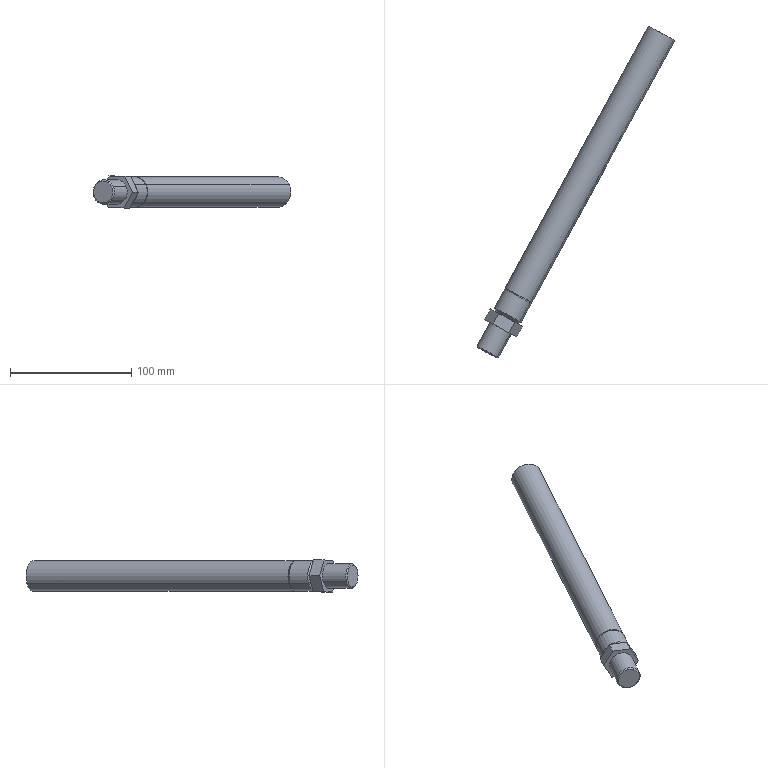Component | SolidWorks | SC-80X130PistonRod-1 | 1 solid | 24 faces | box 162.98 x 273.64 x 26.4 mm | volume 143808 mm3 | plane 12 | cylinder 8 | cone 4 | commonest cylinder face diameters 25 x4 20 x2 23 x2
STEP:
#1=COLOUR_RGB('',0.7922,0.8196,0.9333);
#2=FILL_AREA_STYLE_COLOUR('',#1);
#3=FILL_AREA_STYLE('',(#2));
#4=SURFACE_STYLE_FILL_AREA(#3);
#5=SURFACE_SIDE_STYLE('',(#4));
#6=SURFACE_STYLE_USAGE(.BOTH.,#5);
#7=PRESENTATION_STYLE_ASSIGNMENT((#6));
#8=CARTESIAN_POINT('',(-13.24,0.1934,35.621));
#9=VERTEX_POINT('',#8);
#10=CARTESIAN_POINT('',(-13.848,0.5251,35.246));
#11=VERTEX_POINT('',#10);
#12=CARTESIAN_POINT('',(-13.544,0.3593,35.433));
#13=DIRECTION('',(0.479,0.8778,-0.));
#14=DIRECTION('',(-0.7719,0.4212,-0.4761));
#15=AXIS2_PLACEMENT_3D('',#12,#13,#14);
#16=CIRCLE('',#15,0.3937);
#17=EDGE_CURVE('',#9,#11,#16,.T.);
#18=ORIENTED_EDGE('',*,*,#17,.F.);
#19=CARTESIAN_POINT('',(-13.655,-0.5669,35.621));
#20=VERTEX_POINT('',#19);
#21=CARTESIAN_POINT('',(-13.052,0.539,35.621));
#22=DIRECTION('',(-0.479,-0.8778,0.));
#23=VECTOR('',#22,39.37);
#24=LINE('',#21,#23);
#25=EDGE_CURVE('',#9,#20,#24,.T.);
#26=ORIENTED_EDGE('',*,*,#25,.T.);
#27=CARTESIAN_POINT('',(-14.263,-0.2352,35.246));
#28=VERTEX_POINT('',#27);
#29=CARTESIAN_POINT('',(-13.959,-0.401,35.433));
#30=DIRECTION('',(0.479,0.8778,-0.));
#31=DIRECTION('',(-0.7719,0.4212,-0.4761));
#32=AXIS2_PLACEMENT_3D('',#29,#30,#31);
#33=CIRCLE('',#32,0.3937);
#34=EDGE_CURVE('',#20,#28,#33,.T.);
#35=ORIENTED_EDGE('',*,*,#34,.T.);
#36=CARTESIAN_POINT('',(-13.66,0.8707,35.246));
#37=DIRECTION('',(-0.479,-0.8778,0.));
#38=VECTOR('',#37,39.37);
#39=LINE('',#36,#38);
#40=EDGE_CURVE('',#11,#28,#39,.T.);
#41=ORIENTED_EDGE('',*,*,#40,.F.);
#42=EDGE_LOOP('',(#18,#26,#35,#41));
#43=FACE_OUTER_BOUND('',#42,.T.);
#44=CARTESIAN_POINT('',(-13.356,0.7048,35.433));
#45=DIRECTION('',(-0.479,-0.8778,0.));
#46=DIRECTION('',(-0.7719,0.4212,-0.4761));
#47=AXIS2_PLACEMENT_3D('',#44,#45,#46);
#48=CYLINDRICAL_SURFACE('',#47,0.3937);
#49=ADVANCED_FACE('',(#43),#48,.T.);
#50=CARTESIAN_POINT('',(-14.252,-0.2863,35.264));
#51=VERTEX_POINT('',#50);
#52=CARTESIAN_POINT('',(-13.705,-0.5849,35.602));
#53=VERTEX_POINT('',#52);
#54=CARTESIAN_POINT('',(-13.978,-0.4356,35.433));
#55=DIRECTION('',(-0.479,-0.8778,0.));
#56=DIRECTION('',(-0.7719,0.4212,-0.4761));
#57=AXIS2_PLACEMENT_3D('',#54,#55,#56);
#58=CIRCLE('',#57,0.3543);
#59=EDGE_CURVE('',#51,#53,#58,.T.);
#60=ORIENTED_EDGE('',*,*,#59,.F.);
#61=CARTESIAN_POINT('',(-14.252,-0.2863,35.264));
#62=DIRECTION('',(-0.2071,0.9186,-0.3367));
#63=VECTOR('',#62,39.37);
#64=LINE('',#61,#63);
#65=EDGE_CURVE('',#51,#28,#64,.T.);
#66=ORIENTED_EDGE('',*,*,#65,.T.);
#67=ORIENTED_EDGE('',*,*,#34,.F.);
#68=CARTESIAN_POINT('',(-13.705,-0.5849,35.602));
#69=DIRECTION('',(0.8846,0.3228,0.3367));
#70=VECTOR('',#69,39.37);
#71=LINE('',#68,#70);
#72=EDGE_CURVE('',#53,#20,#71,.T.);
#73=ORIENTED_EDGE('',*,*,#72,.F.);
#74=EDGE_LOOP('',(#60,#66,#67,#73));
#75=FACE_OUTER_BOUND('',#74,.T.);
#76=CARTESIAN_POINT('',(-13.978,-0.4356,35.433));
#77=DIRECTION('',(0.479,0.8778,-0.));
#78=DIRECTION('',(0.7719,-0.4212,0.4761));
#79=AXIS2_PLACEMENT_3D('',#76,#77,#78);
#80=CONICAL_SURFACE('',#79,0.3543,0.7854);
#81=ADVANCED_FACE('',(#75),#80,.T.);
#82=CARTESIAN_POINT('',(-13.34,1.638,35.199));
#83=VERTEX_POINT('',#82);
#84=CARTESIAN_POINT('',(-12.58,1.223,35.667));
#85=VERTEX_POINT('',#84);
#86=CARTESIAN_POINT('',(-12.96,1.431,35.433));
#87=DIRECTION('',(-0.479,-0.8778,0.));
#88=DIRECTION('',(-0.7719,0.4212,-0.4761));
#89=AXIS2_PLACEMENT_3D('',#86,#87,#88);
#90=CIRCLE('',#89,0.4921);
#91=EDGE_CURVE('',#83,#85,#90,.T.);
#92=ORIENTED_EDGE('',*,*,#91,.F.);
#93=CARTESIAN_POINT('',(-8.7,10.139,35.199));
#94=VERTEX_POINT('',#93);
#95=CARTESIAN_POINT('',(-14.358,-0.2283,35.199));
#96=DIRECTION('',(0.479,0.8778,-0.));
#97=VECTOR('',#96,39.37);
#98=LINE('',#95,#97);
#99=EDGE_CURVE('',#83,#94,#98,.T.);
#100=ORIENTED_EDGE('',*,*,#99,.T.);
#101=CARTESIAN_POINT('',(-7.94,9.725,35.667));
#102=VERTEX_POINT('',#101);
#103=CARTESIAN_POINT('',(-8.32,9.932,35.433));
#104=DIRECTION('',(-0.479,-0.8778,0.));
#105=DIRECTION('',(-0.7719,0.4212,-0.4761));
#106=AXIS2_PLACEMENT_3D('',#103,#104,#105);
#107=CIRCLE('',#106,0.4921);
#108=EDGE_CURVE('',#94,#102,#107,.T.);
#109=ORIENTED_EDGE('',*,*,#108,.T.);
#110=CARTESIAN_POINT('',(-13.598,-0.6429,35.667));
#111=DIRECTION('',(0.479,0.8778,-0.));
#112=VECTOR('',#111,39.37);
#113=LINE('',#110,#112);
#114=EDGE_CURVE('',#85,#102,#113,.T.);
#115=ORIENTED_EDGE('',*,*,#114,.F.);
#116=EDGE_LOOP('',(#92,#100,#109,#115));
#117=FACE_OUTER_BOUND('',#116,.T.);
#118=CARTESIAN_POINT('',(-13.978,-0.4356,35.433));
#119=DIRECTION('',(0.479,0.8778,-0.));
#120=DIRECTION('',(0.7719,-0.4212,0.4761));
#121=AXIS2_PLACEMENT_3D('',#118,#119,#120);
#122=CYLINDRICAL_SURFACE('',#121,0.4921);
#123=ADVANCED_FACE('',(#117),#122,.T.);
#124=CARTESIAN_POINT('',(-13.309,1.621,35.218));
#125=VERTEX_POINT('',#124);
#126=CARTESIAN_POINT('',(-12.61,1.24,35.649));
#127=VERTEX_POINT('',#126);
#128=CARTESIAN_POINT('',(-12.96,1.431,35.433));
#129=DIRECTION('',(-0.479,-0.8778,0.));
#130=DIRECTION('',(-0.7719,0.4212,-0.4761));
#131=AXIS2_PLACEMENT_3D('',#128,#129,#130);
#132=CIRCLE('',#131,0.4528);
#133=EDGE_CURVE('',#125,#127,#132,.T.);
#134=ORIENTED_EDGE('',*,*,#133,.T.);
#135=CARTESIAN_POINT('',(-12.629,1.205,35.649));
#136=VERTEX_POINT('',#135);
#137=CARTESIAN_POINT('',(-16.457,-5.81,35.649));
#138=DIRECTION('',(-0.479,-0.8778,0.));
#139=VECTOR('',#138,39.37);
#140=LINE('',#137,#139);
#141=EDGE_CURVE('',#127,#136,#140,.T.);
#142=ORIENTED_EDGE('',*,*,#141,.T.);
#143=CARTESIAN_POINT('',(-13.328,1.587,35.218));
#144=VERTEX_POINT('',#143);
#145=CARTESIAN_POINT('',(-12.978,1.396,35.433));
#146=DIRECTION('',(-0.479,-0.8778,0.));
#147=DIRECTION('',(-0.7719,0.4212,-0.4761));
#148=AXIS2_PLACEMENT_3D('',#145,#146,#147);
#149=CIRCLE('',#148,0.4528);
#150=EDGE_CURVE('',#144,#136,#149,.T.);
#151=ORIENTED_EDGE('',*,*,#150,.F.);
#152=CARTESIAN_POINT('',(-17.156,-5.429,35.218));
#153=DIRECTION('',(-0.479,-0.8778,0.));
#154=VECTOR('',#153,39.37);
#155=LINE('',#152,#154);
#156=EDGE_CURVE('',#125,#144,#155,.T.);
#157=ORIENTED_EDGE('',*,*,#156,.F.);
#158=EDGE_LOOP('',(#134,#142,#151,#157));
#159=FACE_OUTER_BOUND('',#158,.T.);
#160=CARTESIAN_POINT('',(-16.807,-5.619,35.433));
#161=DIRECTION('',(-0.479,-0.8778,0.));
#162=DIRECTION('',(-0.7719,0.4212,-0.4761));
#163=AXIS2_PLACEMENT_3D('',#160,#161,#162);
#164=CYLINDRICAL_SURFACE('',#163,0.4528);
#165=ADVANCED_FACE('',(#159),#164,.T.);
#166=CARTESIAN_POINT('',(-13.66,0.8707,35.246));
#167=VERTEX_POINT('',#166);
#168=CARTESIAN_POINT('',(-13.052,0.539,35.621));
#169=VERTEX_POINT('',#168);
#170=CARTESIAN_POINT('',(-13.356,0.7048,35.433));
#171=DIRECTION('',(-0.479,-0.8778,0.));
#172=DIRECTION('',(-0.7719,0.4212,-0.4761));
#173=AXIS2_PLACEMENT_3D('',#170,#171,#172);
#174=CIRCLE('',#173,0.3937);
#175=EDGE_CURVE('',#167,#169,#174,.T.);
#176=ORIENTED_EDGE('',*,*,#175,.F.);
#177=CARTESIAN_POINT('',(-13.688,0.9985,35.199));
#178=VERTEX_POINT('',#177);
#179=CARTESIAN_POINT('',(-13.66,0.8707,35.246));
#180=DIRECTION('',(-0.2071,0.9186,-0.3367));
#181=VECTOR('',#180,39.37);
#182=LINE('',#179,#181);
#183=EDGE_CURVE('',#167,#178,#182,.T.);
#184=ORIENTED_EDGE('',*,*,#183,.T.);
#185=CARTESIAN_POINT('',(-12.929,0.5839,35.667));
#186=VERTEX_POINT('',#185);
#187=CARTESIAN_POINT('',(-13.309,0.7912,35.433));
#188=DIRECTION('',(0.479,0.8778,-0.));
#189=DIRECTION('',(-0.7719,0.4212,-0.4761));
#190=AXIS2_PLACEMENT_3D('',#187,#188,#189);
#191=CIRCLE('',#190,0.4921);
#192=EDGE_CURVE('',#186,#178,#191,.T.);
#193=ORIENTED_EDGE('',*,*,#192,.F.);
#194=CARTESIAN_POINT('',(-13.052,0.539,35.621));
#195=DIRECTION('',(0.8846,0.3228,0.3367));
#196=VECTOR('',#195,39.37);
#197=LINE('',#194,#196);
#198=EDGE_CURVE('',#169,#186,#197,.T.);
#199=ORIENTED_EDGE('',*,*,#198,.F.);
#200=EDGE_LOOP('',(#176,#184,#193,#199));
#201=FACE_OUTER_BOUND('',#200,.T.);
#202=CARTESIAN_POINT('',(-13.356,0.7048,35.433));
#203=DIRECTION('',(0.479,0.8778,-0.));
#204=DIRECTION('',(0.7719,-0.4212,0.4761));
#205=AXIS2_PLACEMENT_3D('',#202,#203,#204);
#206=CONICAL_SURFACE('',#205,0.3937,0.7854);
#207=ADVANCED_FACE('',(#201),#206,.T.);
#208=ORIENTED_EDGE('',*,*,#192,.T.);
#209=CARTESIAN_POINT('',(-13.358,1.603,35.199));
#210=VERTEX_POINT('',#209);
#211=CARTESIAN_POINT('',(-14.358,-0.2283,35.199));
#212=DIRECTION('',(0.479,0.8778,-0.));
#213=VECTOR('',#212,39.37);
#214=LINE('',#211,#213);
#215=EDGE_CURVE('',#178,#210,#214,.T.);
#216=ORIENTED_EDGE('',*,*,#215,.T.);
#217=CARTESIAN_POINT('',(-12.599,1.189,35.667));
#218=VERTEX_POINT('',#217);
#219=CARTESIAN_POINT('',(-12.978,1.396,35.433));
#220=DIRECTION('',(-0.479,-0.8778,0.));
#221=DIRECTION('',(-0.7719,0.4212,-0.4761));
#222=AXIS2_PLACEMENT_3D('',#219,#220,#221);
#223=CIRCLE('',#222,0.4921);
#224=EDGE_CURVE('',#210,#218,#223,.T.);
#225=ORIENTED_EDGE('',*,*,#224,.T.);
#226=CARTESIAN_POINT('',(-13.598,-0.6429,35.667));
#227=DIRECTION('',(0.479,0.8778,-0.));
#228=VECTOR('',#227,39.37);
#229=LINE('',#226,#228);
#230=EDGE_CURVE('',#186,#218,#229,.T.);
#231=ORIENTED_EDGE('',*,*,#230,.F.);
#232=EDGE_LOOP('',(#208,#216,#225,#231));
#233=FACE_OUTER_BOUND('',#232,.T.);
#234=CARTESIAN_POINT('',(-13.978,-0.4356,35.433));
#235=DIRECTION('',(0.479,0.8778,-0.));
#236=DIRECTION('',(0.7719,-0.4212,0.4761));
#237=AXIS2_PLACEMENT_3D('',#234,#235,#236);
#238=CYLINDRICAL_SURFACE('',#237,0.4921);
#239=ADVANCED_FACE('',(#233),#238,.T.);
#240=ORIENTED_EDGE('',*,*,#215,.F.);
#241=CARTESIAN_POINT('',(-13.309,0.7912,35.433));
#242=DIRECTION('',(0.479,0.8778,-0.));
#243=DIRECTION('',(-0.7719,0.4212,-0.4761));
#244=AXIS2_PLACEMENT_3D('',#241,#242,#243);
#245=CIRCLE('',#244,0.4921);
#246=EDGE_CURVE('',#178,#186,#245,.T.);
#247=ORIENTED_EDGE('',*,*,#246,.T.);
#248=ORIENTED_EDGE('',*,*,#230,.T.);
#249=CARTESIAN_POINT('',(-12.978,1.396,35.433));
#250=DIRECTION('',(-0.479,-0.8778,0.));
#251=DIRECTION('',(-0.7719,0.4212,-0.4761));
#252=AXIS2_PLACEMENT_3D('',#249,#250,#251);
#253=CIRCLE('',#252,0.4921);
#254=EDGE_CURVE('',#218,#210,#253,.T.);
#255=ORIENTED_EDGE('',*,*,#254,.T.);
#256=EDGE_LOOP('',(#240,#247,#248,#255));
#257=FACE_OUTER_BOUND('',#256,.T.);
#258=CARTESIAN_POINT('',(-13.978,-0.4356,35.433));
#259=DIRECTION('',(0.479,0.8778,-0.));
#260=DIRECTION('',(0.7719,-0.4212,0.4761));
#261=AXIS2_PLACEMENT_3D('',#258,#259,#260);
#262=CYLINDRICAL_SURFACE('',#261,0.4921);
#263=ADVANCED_FACE('',(#257),#262,.T.);
#264=ORIENTED_EDGE('',*,*,#183,.F.);
#265=CARTESIAN_POINT('',(-13.356,0.7048,35.433));
#266=DIRECTION('',(-0.479,-0.8778,0.));
#267=DIRECTION('',(-0.7719,0.4212,-0.4761));
#268=AXIS2_PLACEMENT_3D('',#265,#266,#267);
#269=CIRCLE('',#268,0.3937);
#270=EDGE_CURVE('',#169,#167,#269,.T.);
#271=ORIENTED_EDGE('',*,*,#270,.F.);
#272=ORIENTED_EDGE('',*,*,#198,.T.);
#273=ORIENTED_EDGE('',*,*,#246,.F.);
#274=EDGE_LOOP('',(#264,#271,#272,#273));
#275=FACE_OUTER_BOUND('',#274,.T.);
#276=CARTESIAN_POINT('',(-13.356,0.7048,35.433));
#277=DIRECTION('',(0.479,0.8778,-0.));
#278=DIRECTION('',(0.7719,-0.4212,0.4761));
#279=AXIS2_PLACEMENT_3D('',#276,#277,#278);
#280=CONICAL_SURFACE('',#279,0.3937,0.7854);
#281=ADVANCED_FACE('',(#275),#280,.T.);
#282=ORIENTED_EDGE('',*,*,#150,.T.);
#283=CARTESIAN_POINT('',(-12.978,1.396,35.433));
#284=DIRECTION('',(-0.479,-0.8778,0.));
#285=DIRECTION('',(-0.7719,0.4212,-0.4761));
#286=AXIS2_PLACEMENT_3D('',#283,#284,#285);
#287=CIRCLE('',#286,0.4528);
#288=EDGE_CURVE('',#136,#144,#287,.T.);
#289=ORIENTED_EDGE('',*,*,#288,.T.);
#290=EDGE_LOOP('',(#282,#289));
#291=FACE_BOUND('',#290,.T.);
#292=ORIENTED_EDGE('',*,*,#254,.F.);
#293=ORIENTED_EDGE('',*,*,#224,.F.);
#294=EDGE_LOOP('',(#292,#293));
#295=FACE_OUTER_BOUND('',#294,.T.);
#296=CARTESIAN_POINT('',(-12.773,1.284,35.));
#297=DIRECTION('',(0.479,0.8778,-0.));
#298=DIRECTION('',(0.7719,-0.4212,0.4761));
#299=AXIS2_PLACEMENT_3D('',#296,#297,#298);
#300=PLANE('',#299);
#301=ADVANCED_FACE('',(#291,#295),#300,.T.);
#302=CARTESIAN_POINT('',(-12.96,1.431,35.433));
#303=DIRECTION('',(-0.479,-0.8778,0.));
#304=DIRECTION('',(-0.7719,0.4212,-0.4761));
#305=AXIS2_PLACEMENT_3D('',#302,#303,#304);
#306=CIRCLE('',#305,0.4921);
#307=EDGE_CURVE('',#85,#83,#306,.T.);
#308=ORIENTED_EDGE('',*,*,#307,.T.);
#309=ORIENTED_EDGE('',*,*,#91,.T.);
#310=EDGE_LOOP('',(#308,#309));
#311=FACE_OUTER_BOUND('',#310,.T.);
#312=ORIENTED_EDGE('',*,*,#133,.F.);
#313=CARTESIAN_POINT('',(-12.96,1.431,35.433));
#314=DIRECTION('',(-0.479,-0.8778,0.));
#315=DIRECTION('',(-0.7719,0.4212,-0.4761));
#316=AXIS2_PLACEMENT_3D('',#313,#314,#315);
#317=CIRCLE('',#316,0.4528);
#318=EDGE_CURVE('',#127,#125,#317,.T.);
#319=ORIENTED_EDGE('',*,*,#318,.F.);
#320=EDGE_LOOP('',(#312,#319));
#321=FACE_BOUND('',#320,.T.);
#322=CARTESIAN_POINT('',(-12.754,1.318,35.));
#323=DIRECTION('',(-0.479,-0.8778,0.));
#324=DIRECTION('',(-0.7719,0.4212,-0.4761));
#325=AXIS2_PLACEMENT_3D('',#322,#323,#324);
#326=PLANE('',#325);
#327=ADVANCED_FACE('',(#311,#321),#326,.T.);
#328=ORIENTED_EDGE('',*,*,#141,.F.);
#329=ORIENTED_EDGE('',*,*,#318,.T.);
#330=ORIENTED_EDGE('',*,*,#156,.T.);
#331=ORIENTED_EDGE('',*,*,#288,.F.);
#332=EDGE_LOOP('',(#328,#329,#330,#331));
#333=FACE_OUTER_BOUND('',#332,.T.);
#334=CARTESIAN_POINT('',(-16.807,-5.619,35.433));
#335=DIRECTION('',(-0.479,-0.8778,0.));
#336=DIRECTION('',(-0.7719,0.4212,-0.4761));
#337=AXIS2_PLACEMENT_3D('',#334,#335,#336);
#338=CYLINDRICAL_SURFACE('',#337,0.4528);
#339=ADVANCED_FACE('',(#333),#338,.T.);
#340=CARTESIAN_POINT('',(-8.32,9.932,35.433));
#341=DIRECTION('',(-0.479,-0.8778,0.));
#342=DIRECTION('',(-0.7719,0.4212,-0.4761));
#343=AXIS2_PLACEMENT_3D('',#340,#341,#342);
#344=CIRCLE('',#343,0.4921);
#345=EDGE_CURVE('',#102,#94,#344,.T.);
#346=ORIENTED_EDGE('',*,*,#345,.F.);
#347=ORIENTED_EDGE('',*,*,#108,.F.);
#348=EDGE_LOOP('',(#346,#347));
#349=FACE_OUTER_BOUND('',#348,.T.);
#350=CARTESIAN_POINT('',(-8.32,9.932,35.433));
#351=DIRECTION('',(-0.479,-0.8778,0.));
#352=DIRECTION('',(-0.7719,0.4212,-0.4761));
#353=AXIS2_PLACEMENT_3D('',#350,#351,#352);
#354=PLANE('',#353);
#355=ADVANCED_FACE('',(#349),#354,.F.);
#356=ORIENTED_EDGE('',*,*,#99,.F.);
#357=ORIENTED_EDGE('',*,*,#307,.F.);
#358=ORIENTED_EDGE('',*,*,#114,.T.);
#359=ORIENTED_EDGE('',*,*,#345,.T.);
#360=EDGE_LOOP('',(#356,#357,#358,#359));
#361=FACE_OUTER_BOUND('',#360,.T.);
#362=CARTESIAN_POINT('',(-13.978,-0.4356,35.433));
#363=DIRECTION('',(0.479,0.8778,-0.));
#364=DIRECTION('',(0.7719,-0.4212,0.4761));
#365=AXIS2_PLACEMENT_3D('',#362,#363,#364);
#366=CYLINDRICAL_SURFACE('',#365,0.4921);
#367=ADVANCED_FACE('',(#361),#366,.T.);
#368=CARTESIAN_POINT('',(-13.084,0.5566,35.937));
#369=VERTEX_POINT('',#368);
#370=CARTESIAN_POINT('',(-13.603,0.8396,35.953));
#371=VERTEX_POINT('',#370);
#372=CARTESIAN_POINT('',(-13.084,0.5566,35.937));
#373=DIRECTION('',(-0.8775,0.4789,0.02735));
#374=VECTOR('',#373,39.37);
#375=LINE('',#372,#374);
#376=EDGE_CURVE('',#369,#371,#375,.T.);
#377=ORIENTED_EDGE('',*,*,#376,.T.);
#378=CARTESIAN_POINT('',(-13.791,0.494,35.953));
#379=VERTEX_POINT('',#378);
#380=CARTESIAN_POINT('',(-13.791,0.494,35.953));
#381=DIRECTION('',(0.479,0.8778,-0.));
#382=VECTOR('',#381,39.37);
#383=LINE('',#380,#382);
#384=EDGE_CURVE('',#379,#371,#383,.T.);
#385=ORIENTED_EDGE('',*,*,#384,.F.);
#386=CARTESIAN_POINT('',(-13.273,0.211,35.937));
#387=VERTEX_POINT('',#386);
#388=CARTESIAN_POINT('',(-13.273,0.211,35.937));
#389=DIRECTION('',(-0.8775,0.4789,0.02735));
#390=VECTOR('',#389,39.37);
#391=LINE('',#388,#390);
#392=EDGE_CURVE('',#387,#379,#391,.T.);
#393=ORIENTED_EDGE('',*,*,#392,.F.);
#394=CARTESIAN_POINT('',(-13.273,0.211,35.937));
#395=DIRECTION('',(0.479,0.8778,-0.));
#396=VECTOR('',#395,39.37);
#397=LINE('',#394,#396);
#398=EDGE_CURVE('',#387,#369,#397,.T.);
#399=ORIENTED_EDGE('',*,*,#398,.T.);
#400=EDGE_LOOP('',(#377,#385,#393,#399));
#401=FACE_OUTER_BOUND('',#400,.T.);
#402=CARTESIAN_POINT('',(-13.273,0.211,35.937));
#403=DIRECTION('',(-0.02401,0.0131,-0.9996));
#404=DIRECTION('',(0.8775,-0.4789,-0.02735));
#405=AXIS2_PLACEMENT_3D('',#402,#403,#404);
#406=PLANE('',#405);
#407=ADVANCED_FACE('',(#401),#406,.F.);
#408=CARTESIAN_POINT('',(-13.874,0.9878,35.449));
#409=VERTEX_POINT('',#408);
#410=CARTESIAN_POINT('',(-13.603,0.8396,35.953));
#411=DIRECTION('',(-0.4595,0.2508,-0.852));
#412=VECTOR('',#411,39.37);
#413=LINE('',#410,#412);
#414=EDGE_CURVE('',#371,#409,#413,.T.);
#415=ORIENTED_EDGE('',*,*,#414,.T.);
#416=CARTESIAN_POINT('',(-14.063,0.6422,35.449));
#417=VERTEX_POINT('',#416);
#418=CARTESIAN_POINT('',(-14.063,0.6422,35.449));
#419=DIRECTION('',(0.479,0.8778,-0.));
#420=VECTOR('',#419,39.37);
#421=LINE('',#418,#420);
#422=EDGE_CURVE('',#417,#409,#421,.T.);
#423=ORIENTED_EDGE('',*,*,#422,.F.);
#424=CARTESIAN_POINT('',(-13.791,0.494,35.953));
#425=DIRECTION('',(-0.4595,0.2508,-0.852));
#426=VECTOR('',#425,39.37);
#427=LINE('',#424,#426);
#428=EDGE_CURVE('',#379,#417,#427,.T.);
#429=ORIENTED_EDGE('',*,*,#428,.F.);
#430=ORIENTED_EDGE('',*,*,#384,.T.);
#431=EDGE_LOOP('',(#415,#423,#429,#430));
#432=FACE_OUTER_BOUND('',#431,.T.);
#433=CARTESIAN_POINT('',(-13.791,0.494,35.953));
#434=DIRECTION('',(0.7479,-0.4081,-0.5235));
#435=DIRECTION('',(0.4595,-0.2508,0.852));
#436=AXIS2_PLACEMENT_3D('',#433,#434,#435);
#437=PLANE('',#436);
#438=ADVANCED_FACE('',(#432),#437,.F.);
#439=CARTESIAN_POINT('',(-13.627,0.853,34.93));
#440=VERTEX_POINT('',#439);
#441=CARTESIAN_POINT('',(-13.874,0.9878,35.449));
#442=DIRECTION('',(0.4179,-0.2281,-0.8794));
#443=VECTOR('',#442,39.37);
#444=LINE('',#441,#443);
#445=EDGE_CURVE('',#409,#440,#444,.T.);
#446=ORIENTED_EDGE('',*,*,#445,.T.);
#447=CARTESIAN_POINT('',(-13.816,0.5075,34.93));
#448=VERTEX_POINT('',#447);
#449=CARTESIAN_POINT('',(-13.816,0.5075,34.93));
#450=DIRECTION('',(0.479,0.8778,-0.));
#451=VECTOR('',#450,39.37);
#452=LINE('',#449,#451);
#453=EDGE_CURVE('',#448,#440,#452,.T.);
#454=ORIENTED_EDGE('',*,*,#453,.F.);
#455=CARTESIAN_POINT('',(-14.063,0.6422,35.449));
#456=DIRECTION('',(0.4179,-0.2281,-0.8794));
#457=VECTOR('',#456,39.37);
#458=LINE('',#455,#457);
#459=EDGE_CURVE('',#417,#448,#458,.T.);
#460=ORIENTED_EDGE('',*,*,#459,.F.);
#461=ORIENTED_EDGE('',*,*,#422,.T.);
#462=EDGE_LOOP('',(#446,#454,#460,#461));
#463=FACE_OUTER_BOUND('',#462,.T.);
#464=CARTESIAN_POINT('',(-14.063,0.6422,35.449));
#465=DIRECTION('',(0.7719,-0.4212,0.4761));
#466=DIRECTION('',(-0.4179,0.2281,0.8794));
#467=AXIS2_PLACEMENT_3D('',#464,#465,#466);
#468=PLANE('',#467);
#469=ADVANCED_FACE('',(#463),#468,.F.);
#470=CARTESIAN_POINT('',(-13.109,0.57,34.913));
#471=VERTEX_POINT('',#470);
#472=CARTESIAN_POINT('',(-13.627,0.853,34.93));
#473=DIRECTION('',(0.8775,-0.4789,-0.02735));
#474=VECTOR('',#473,39.37);
#475=LINE('',#472,#474);
#476=EDGE_CURVE('',#440,#471,#475,.T.);
#477=ORIENTED_EDGE('',*,*,#476,.T.);
#478=CARTESIAN_POINT('',(-13.297,0.2245,34.913));
#479=VERTEX_POINT('',#478);
#480=CARTESIAN_POINT('',(-13.297,0.2245,34.913));
#481=DIRECTION('',(0.479,0.8778,-0.));
#482=VECTOR('',#481,39.37);
#483=LINE('',#480,#482);
#484=EDGE_CURVE('',#479,#471,#483,.T.);
#485=ORIENTED_EDGE('',*,*,#484,.F.);
#486=CARTESIAN_POINT('',(-13.816,0.5075,34.93));
#487=DIRECTION('',(0.8775,-0.4789,-0.02735));
#488=VECTOR('',#487,39.37);
#489=LINE('',#486,#488);
#490=EDGE_CURVE('',#448,#479,#489,.T.);
#491=ORIENTED_EDGE('',*,*,#490,.F.);
#492=ORIENTED_EDGE('',*,*,#453,.T.);
#493=EDGE_LOOP('',(#477,#485,#491,#492));
#494=FACE_OUTER_BOUND('',#493,.T.);
#495=CARTESIAN_POINT('',(-13.816,0.5075,34.93));
#496=DIRECTION('',(0.02401,-0.0131,0.9996));
#497=DIRECTION('',(-0.8775,0.4789,0.02735));
#498=AXIS2_PLACEMENT_3D('',#495,#496,#497);
#499=PLANE('',#498);
#500=ADVANCED_FACE('',(#494),#499,.F.);
#501=CARTESIAN_POINT('',(-12.837,0.4218,35.417));
#502=VERTEX_POINT('',#501);
#503=CARTESIAN_POINT('',(-13.109,0.57,34.913));
#504=DIRECTION('',(0.4595,-0.2508,0.852));
#505=VECTOR('',#504,39.37);
#506=LINE('',#503,#505);
#507=EDGE_CURVE('',#471,#502,#506,.T.);
#508=ORIENTED_EDGE('',*,*,#507,.T.);
#509=CARTESIAN_POINT('',(-13.026,0.07626,35.417));
#510=VERTEX_POINT('',#509);
#511=CARTESIAN_POINT('',(-13.026,0.07626,35.417));
#512=DIRECTION('',(0.479,0.8778,-0.));
#513=VECTOR('',#512,39.37);
#514=LINE('',#511,#513);
#515=EDGE_CURVE('',#510,#502,#514,.T.);
#516=ORIENTED_EDGE('',*,*,#515,.F.);
#517=CARTESIAN_POINT('',(-13.297,0.2245,34.913));
#518=DIRECTION('',(0.4595,-0.2508,0.852));
#519=VECTOR('',#518,39.37);
#520=LINE('',#517,#519);
#521=EDGE_CURVE('',#479,#510,#520,.T.);
#522=ORIENTED_EDGE('',*,*,#521,.F.);
#523=ORIENTED_EDGE('',*,*,#484,.T.);
#524=EDGE_LOOP('',(#508,#516,#522,#523));
#525=FACE_OUTER_BOUND('',#524,.T.);
#526=CARTESIAN_POINT('',(-13.297,0.2245,34.913));
#527=DIRECTION('',(-0.7479,0.4081,0.5235));
#528=DIRECTION('',(-0.4595,0.2508,-0.852));
#529=AXIS2_PLACEMENT_3D('',#526,#527,#528);
#530=PLANE('',#529);
#531=ADVANCED_FACE('',(#525),#530,.F.);
#532=CARTESIAN_POINT('',(-12.837,0.4218,35.417));
#533=DIRECTION('',(-0.4179,0.2281,0.8794));
#534=VECTOR('',#533,39.37);
#535=LINE('',#532,#534);
#536=EDGE_CURVE('',#502,#369,#535,.T.);
#537=ORIENTED_EDGE('',*,*,#536,.T.);
#538=ORIENTED_EDGE('',*,*,#398,.F.);
#539=CARTESIAN_POINT('',(-13.026,0.07626,35.417));
#540=DIRECTION('',(-0.4179,0.2281,0.8794));
#541=VECTOR('',#540,39.37);
#542=LINE('',#539,#541);
#543=EDGE_CURVE('',#510,#387,#542,.T.);
#544=ORIENTED_EDGE('',*,*,#543,.F.);
#545=ORIENTED_EDGE('',*,*,#515,.T.);
#546=EDGE_LOOP('',(#537,#538,#544,#545));
#547=FACE_OUTER_BOUND('',#546,.T.);
#548=CARTESIAN_POINT('',(-13.026,0.07626,35.417));
#549=DIRECTION('',(-0.7719,0.4212,-0.4761));
#550=DIRECTION('',(0.4179,-0.2281,-0.8794));
#551=AXIS2_PLACEMENT_3D('',#548,#549,#550);
#552=PLANE('',#551);
#553=ADVANCED_FACE('',(#547),#552,.F.);
#554=CARTESIAN_POINT('',(-13.544,0.3593,35.433));
#555=DIRECTION('',(0.479,0.8778,-0.));
#556=DIRECTION('',(-0.7719,0.4212,-0.4761));
#557=AXIS2_PLACEMENT_3D('',#554,#555,#556);
#558=CIRCLE('',#557,0.3937);
#559=EDGE_CURVE('',#11,#9,#558,.T.);
#560=ORIENTED_EDGE('',*,*,#559,.T.);
#561=ORIENTED_EDGE('',*,*,#17,.T.);
#562=EDGE_LOOP('',(#560,#561));
#563=FACE_BOUND('',#562,.T.);
#564=ORIENTED_EDGE('',*,*,#392,.T.);
#565=ORIENTED_EDGE('',*,*,#428,.T.);
#566=ORIENTED_EDGE('',*,*,#459,.T.);
#567=ORIENTED_EDGE('',*,*,#490,.T.);
#568=ORIENTED_EDGE('',*,*,#521,.T.);
#569=ORIENTED_EDGE('',*,*,#543,.T.);
#570=EDGE_LOOP('',(#564,#565,#566,#567,#568,#569));
#571=FACE_OUTER_BOUND('',#570,.T.);
#572=CARTESIAN_POINT('',(-13.544,0.3593,35.433));
#573=DIRECTION('',(-0.479,-0.8778,0.));
#574=DIRECTION('',(-0.7719,0.4212,-0.4761));
#575=AXIS2_PLACEMENT_3D('',#572,#573,#574);
#576=PLANE('',#575);
#577=ADVANCED_FACE('',(#563,#571),#576,.T.);
#578=ORIENTED_EDGE('',*,*,#270,.T.);
#579=ORIENTED_EDGE('',*,*,#175,.T.);
#580=EDGE_LOOP('',(#578,#579));
#581=FACE_BOUND('',#580,.T.);
#582=ORIENTED_EDGE('',*,*,#376,.F.);
#583=ORIENTED_EDGE('',*,*,#536,.F.);
#584=ORIENTED_EDGE('',*,*,#507,.F.);
#585=ORIENTED_EDGE('',*,*,#476,.F.);
#586=ORIENTED_EDGE('',*,*,#445,.F.);
#587=ORIENTED_EDGE('',*,*,#414,.F.);
#588=EDGE_LOOP('',(#582,#583,#584,#585,#586,#587));
#589=FACE_OUTER_BOUND('',#588,.T.);
#590=CARTESIAN_POINT('',(-13.356,0.7048,35.433));
#591=DIRECTION('',(-0.479,-0.8778,0.));
#592=DIRECTION('',(-0.7719,0.4212,-0.4761));
#593=AXIS2_PLACEMENT_3D('',#590,#591,#592);
#594=PLANE('',#593);
#595=ADVANCED_FACE('',(#581,#589),#594,.F.);
#596=CARTESIAN_POINT('',(-13.978,-0.4356,35.433));
#597=DIRECTION('',(-0.479,-0.8778,0.));
#598=DIRECTION('',(-0.7719,0.4212,-0.4761));
#599=AXIS2_PLACEMENT_3D('',#596,#597,#598);
#600=CIRCLE('',#599,0.3543);
#601=EDGE_CURVE('',#53,#51,#600,.T.);
#602=ORIENTED_EDGE('',*,*,#601,.T.);
#603=ORIENTED_EDGE('',*,*,#59,.T.);
#604=EDGE_LOOP('',(#602,#603));
#605=FACE_OUTER_BOUND('',#604,.T.);
#606=CARTESIAN_POINT('',(-13.978,-0.4356,35.433));
#607=DIRECTION('',(-0.479,-0.8778,0.));
#608=DIRECTION('',(-0.7719,0.4212,-0.4761));
#609=AXIS2_PLACEMENT_3D('',#606,#607,#608);
#610=PLANE('',#609);
#611=ADVANCED_FACE('',(#605),#610,.T.);
#612=ORIENTED_EDGE('',*,*,#65,.F.);
#613=ORIENTED_EDGE('',*,*,#601,.F.);
#614=ORIENTED_EDGE('',*,*,#72,.T.);
#615=CARTESIAN_POINT('',(-13.959,-0.401,35.433));
#616=DIRECTION('',(0.479,0.8778,-0.));
#617=DIRECTION('',(-0.7719,0.4212,-0.4761));
#618=AXIS2_PLACEMENT_3D('',#615,#616,#617);
#619=CIRCLE('',#618,0.3937);
#620=EDGE_CURVE('',#28,#20,#619,.T.);
#621=ORIENTED_EDGE('',*,*,#620,.F.);
#622=EDGE_LOOP('',(#612,#613,#614,#621));
#623=FACE_OUTER_BOUND('',#622,.T.);
#624=CARTESIAN_POINT('',(-13.978,-0.4356,35.433));
#625=DIRECTION('',(0.479,0.8778,-0.));
#626=DIRECTION('',(0.7719,-0.4212,0.4761));
#627=AXIS2_PLACEMENT_3D('',#624,#625,#626);
#628=CONICAL_SURFACE('',#627,0.3543,0.7854);
#629=ADVANCED_FACE('',(#623),#628,.T.);
#630=ORIENTED_EDGE('',*,*,#25,.F.);
#631=ORIENTED_EDGE('',*,*,#559,.F.);
#632=ORIENTED_EDGE('',*,*,#40,.T.);
#633=ORIENTED_EDGE('',*,*,#620,.T.);
#634=EDGE_LOOP('',(#630,#631,#632,#633));
#635=FACE_OUTER_BOUND('',#634,.T.);
#636=CARTESIAN_POINT('',(-13.356,0.7048,35.433));
#637=DIRECTION('',(-0.479,-0.8778,0.));
#638=DIRECTION('',(-0.7719,0.4212,-0.4761));
#639=AXIS2_PLACEMENT_3D('',#636,#637,#638);
#640=CYLINDRICAL_SURFACE('',#639,0.3937);
#641=ADVANCED_FACE('',(#635),#640,.T.);
#642=CLOSED_SHELL('',(#49,#81,#123,#165,#207,#239,#263,#281,#301,#327,#339,#355,#367,#407,#438,#469,#500,#531,#553,#577,#595,#611,#629,#641));
#643=MANIFOLD_SOLID_BREP('',#642);
#644=STYLED_ITEM('',(#7),#643);
#645=(LENGTH_UNIT()NAMED_UNIT(*)SI_UNIT($,.METRE.));
#646=LENGTH_MEASURE_WITH_UNIT(LENGTH_MEASURE(0.0254),#645);
#647=DIMENSIONAL_EXPONENTS(1.,0.,0.,0.,0.,0.,0.);
#648=(CONVERSION_BASED_UNIT('',#646)LENGTH_UNIT()NAMED_UNIT(#647));
#649=UNCERTAINTY_MEASURE_WITH_UNIT(LENGTH_MEASURE(0.00001),#648,'','');
#650=(NAMED_UNIT(*)PLANE_ANGLE_UNIT()SI_UNIT($,.RADIAN.));
#651=(NAMED_UNIT(*)SI_UNIT($,.STERADIAN.)SOLID_ANGLE_UNIT());
#652=(GEOMETRIC_REPRESENTATION_CONTEXT(3)GLOBAL_UNCERTAINTY_ASSIGNED_CONTEXT((#649))GLOBAL_UNIT_ASSIGNED_CONTEXT((#648,#650,#651))REPRESENTATION_CONTEXT('',''));
#653=MECHANICAL_DESIGN_GEOMETRIC_PRESENTATION_REPRESENTATION('',(#644),#652);
#654=PRESENTATION_LAYER_ASSIGNMENT('','',(#644));
#655=CARTESIAN_POINT('',(0.,0.,0.));
#656=DIRECTION('',(0.,0.,1.));
#657=DIRECTION('',(1.,0.,0.));
#658=AXIS2_PLACEMENT_3D('',#655,#656,#657);
#659=(LENGTH_UNIT()NAMED_UNIT(*)SI_UNIT($,.METRE.));
#660=LENGTH_MEASURE_WITH_UNIT(LENGTH_MEASURE(0.0254),#659);
#661=DIMENSIONAL_EXPONENTS(1.,0.,0.,0.,0.,0.,0.);
#662=(CONVERSION_BASED_UNIT('',#660)LENGTH_UNIT()NAMED_UNIT(#661));
#663=UNCERTAINTY_MEASURE_WITH_UNIT(LENGTH_MEASURE(0.00001),#662,'','');
#664=(NAMED_UNIT(*)PLANE_ANGLE_UNIT()SI_UNIT($,.RADIAN.));
#665=(NAMED_UNIT(*)SI_UNIT($,.STERADIAN.)SOLID_ANGLE_UNIT());
#666=(GEOMETRIC_REPRESENTATION_CONTEXT(3)GLOBAL_UNCERTAINTY_ASSIGNED_CONTEXT((#663))GLOBAL_UNIT_ASSIGNED_CONTEXT((#662,#664,#665))REPRESENTATION_CONTEXT('',''));
#667=ADVANCED_BREP_SHAPE_REPRESENTATION('',(#643,#658),#666);